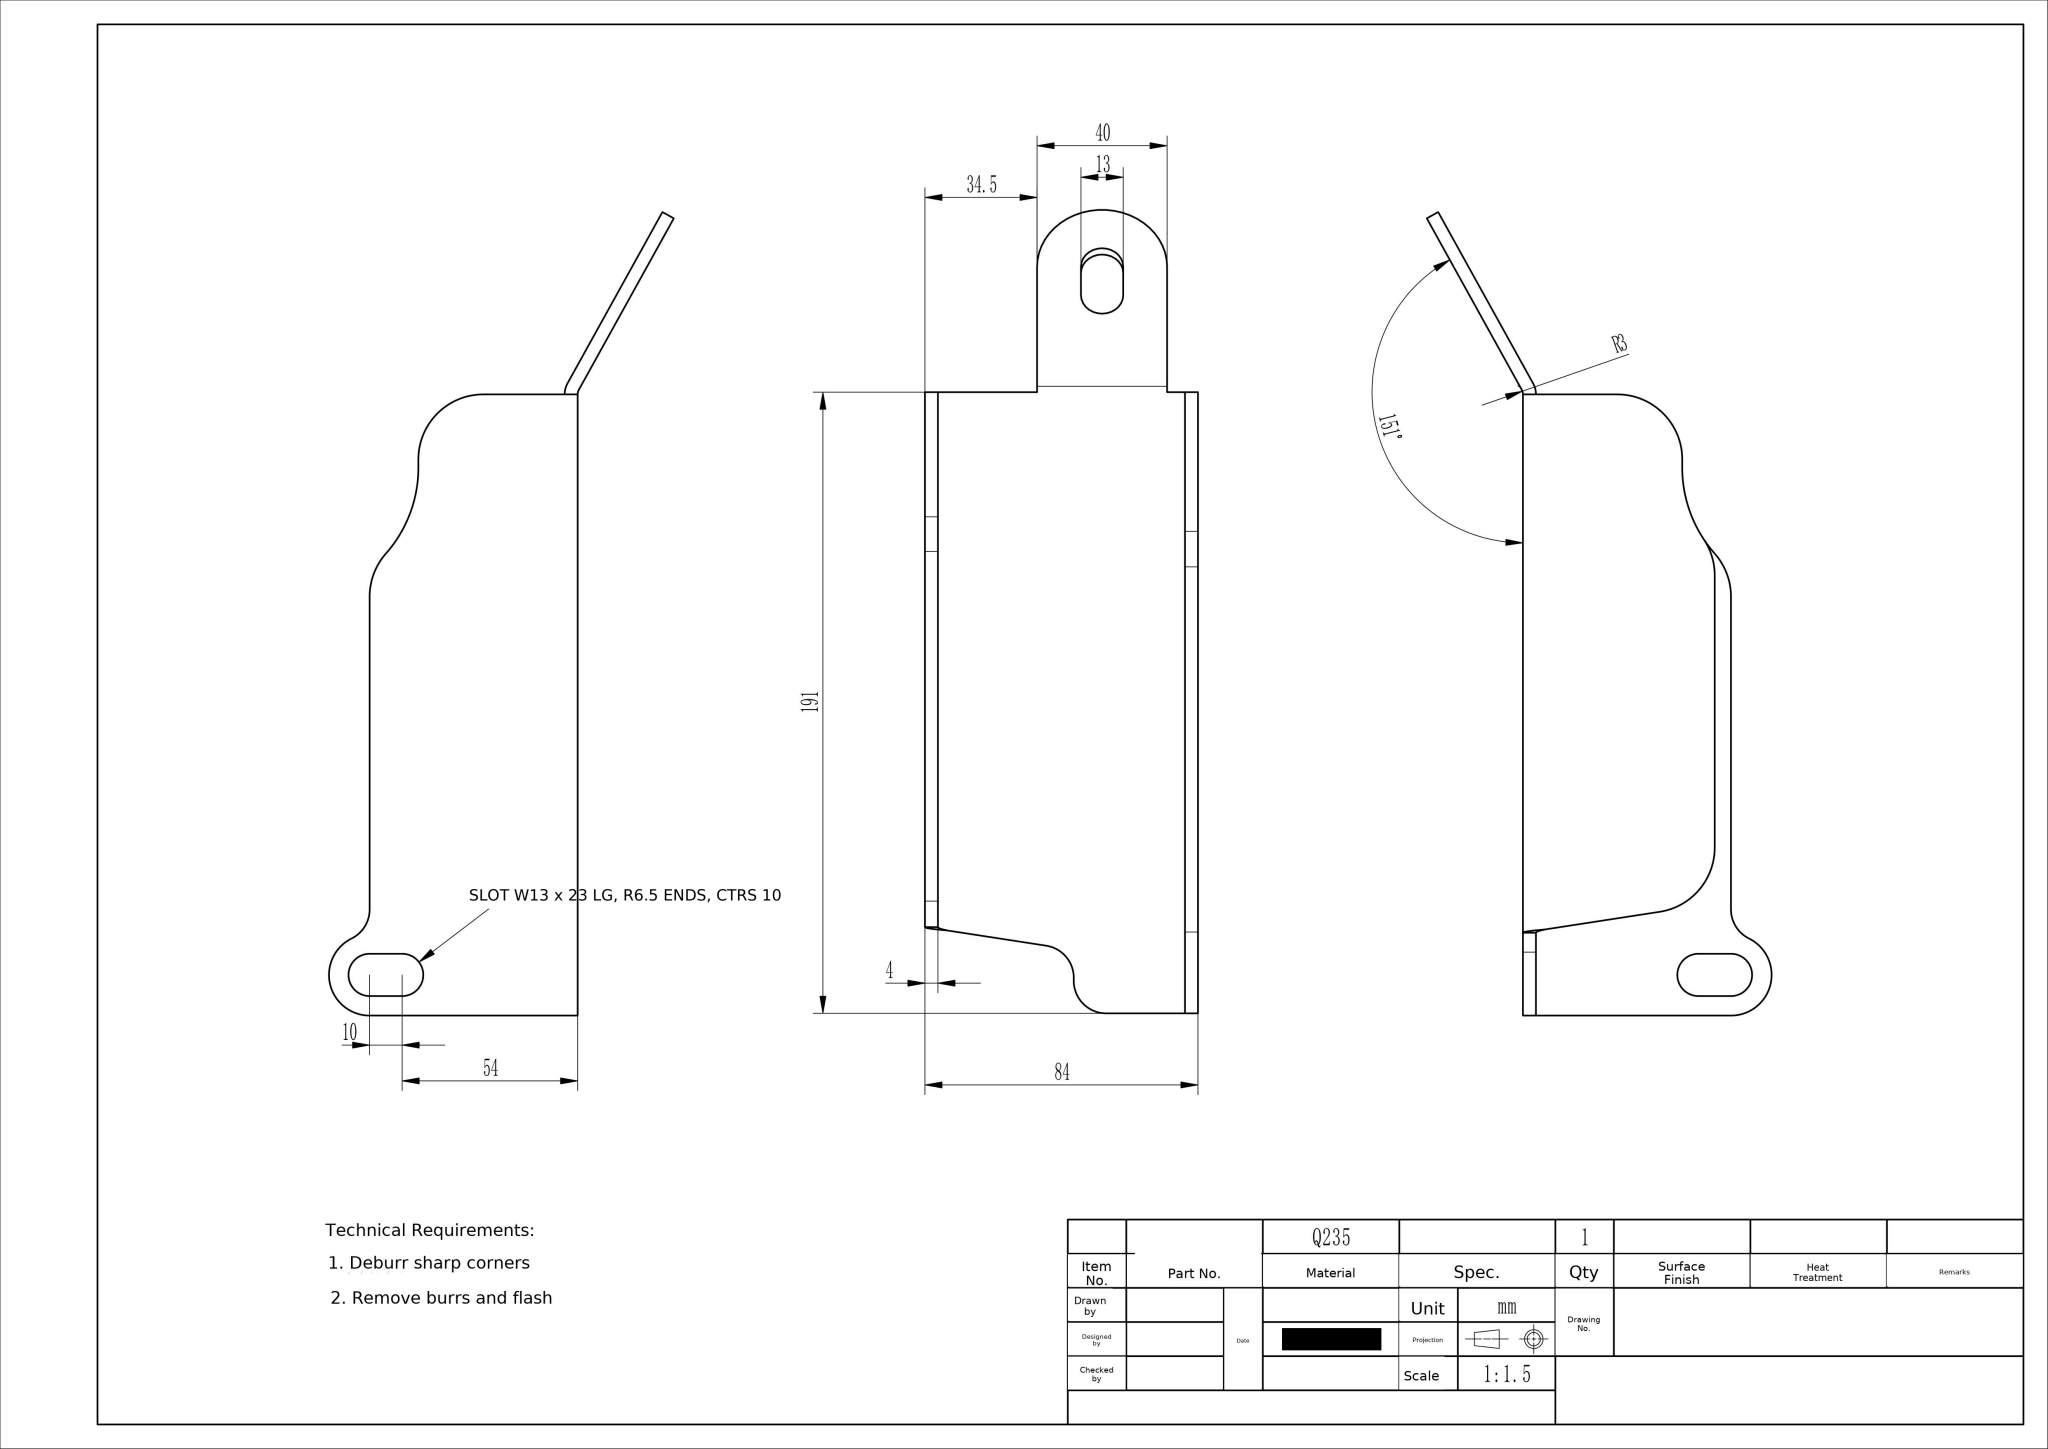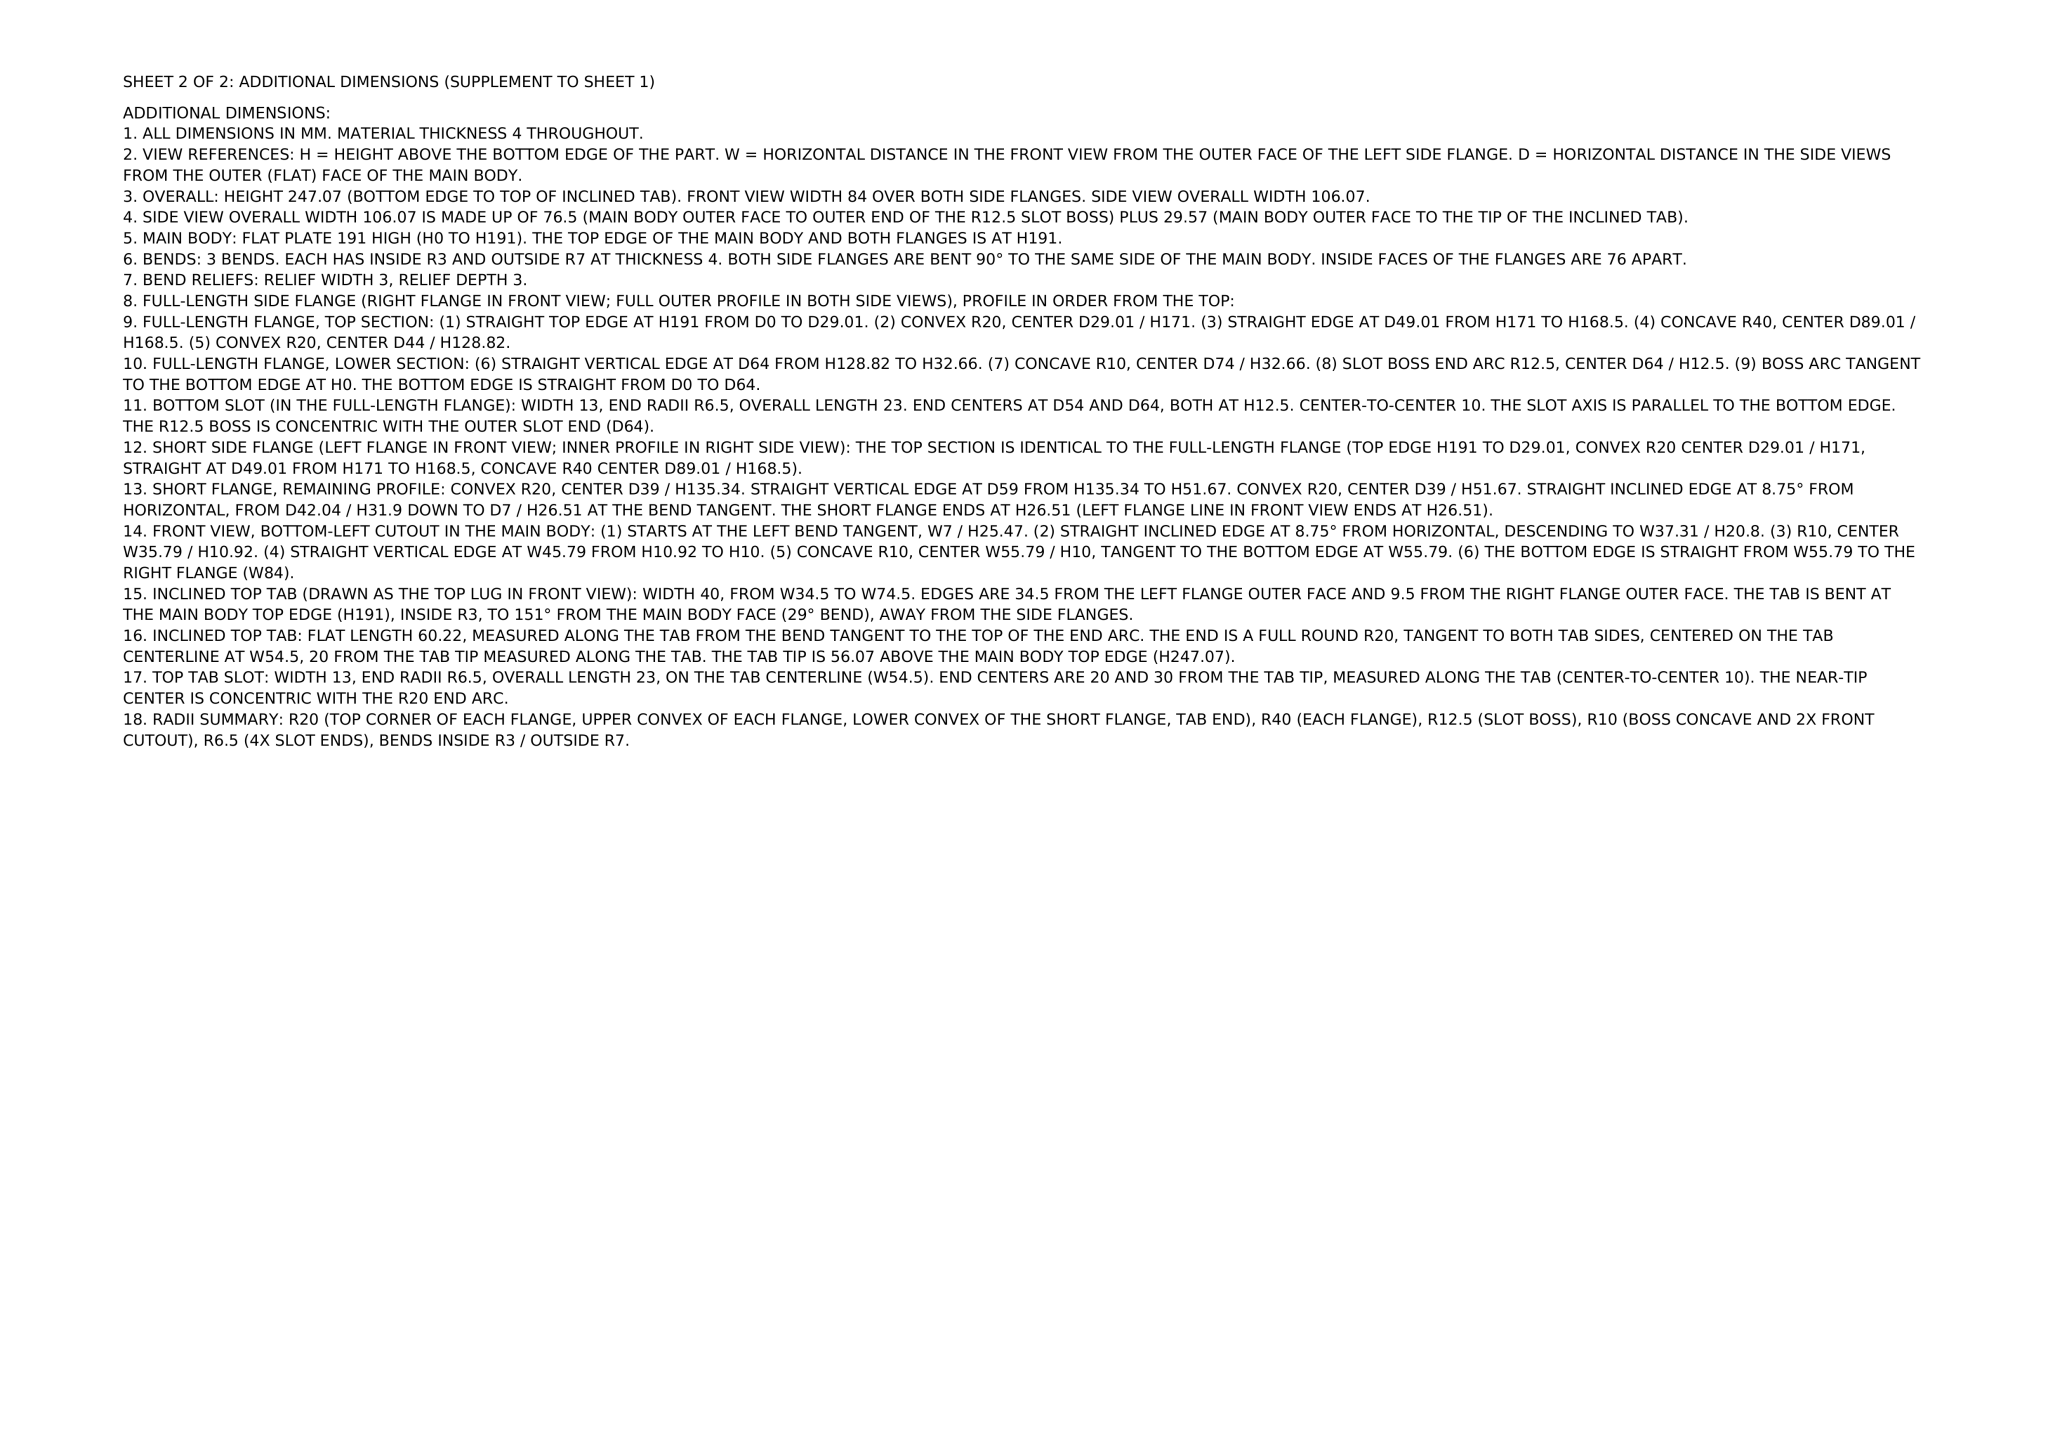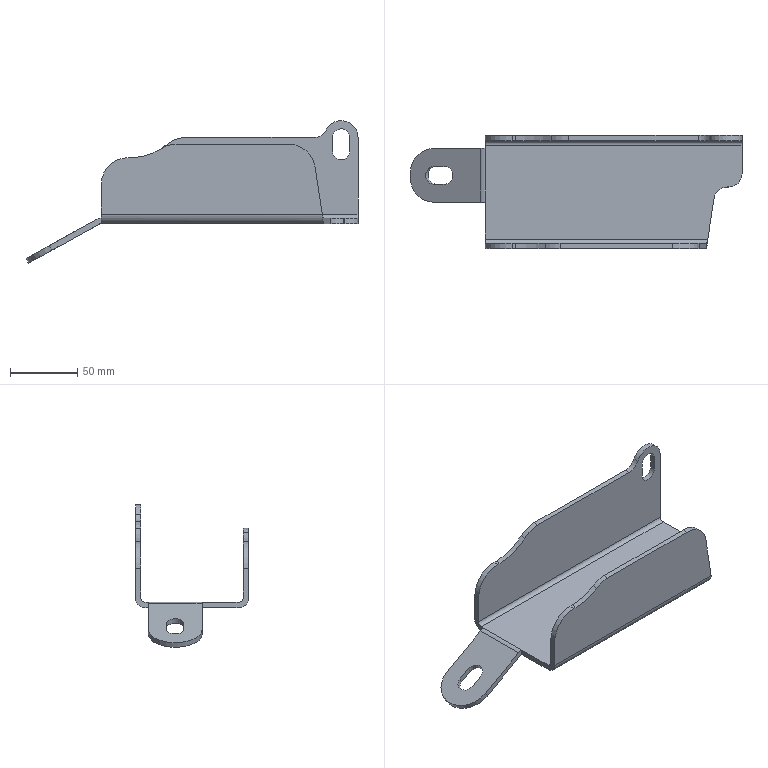Part | NX | mm | 1 solid | 47 faces | box 247.07 x 84 x 106.07 mm | volume 141099 mm3 | plane 24 | cylinder 22 | spline 1 | commonest cylinder face diameters 40 x6 13 x4 14 x3 6 x3 20 x3 80 x2 25 x1